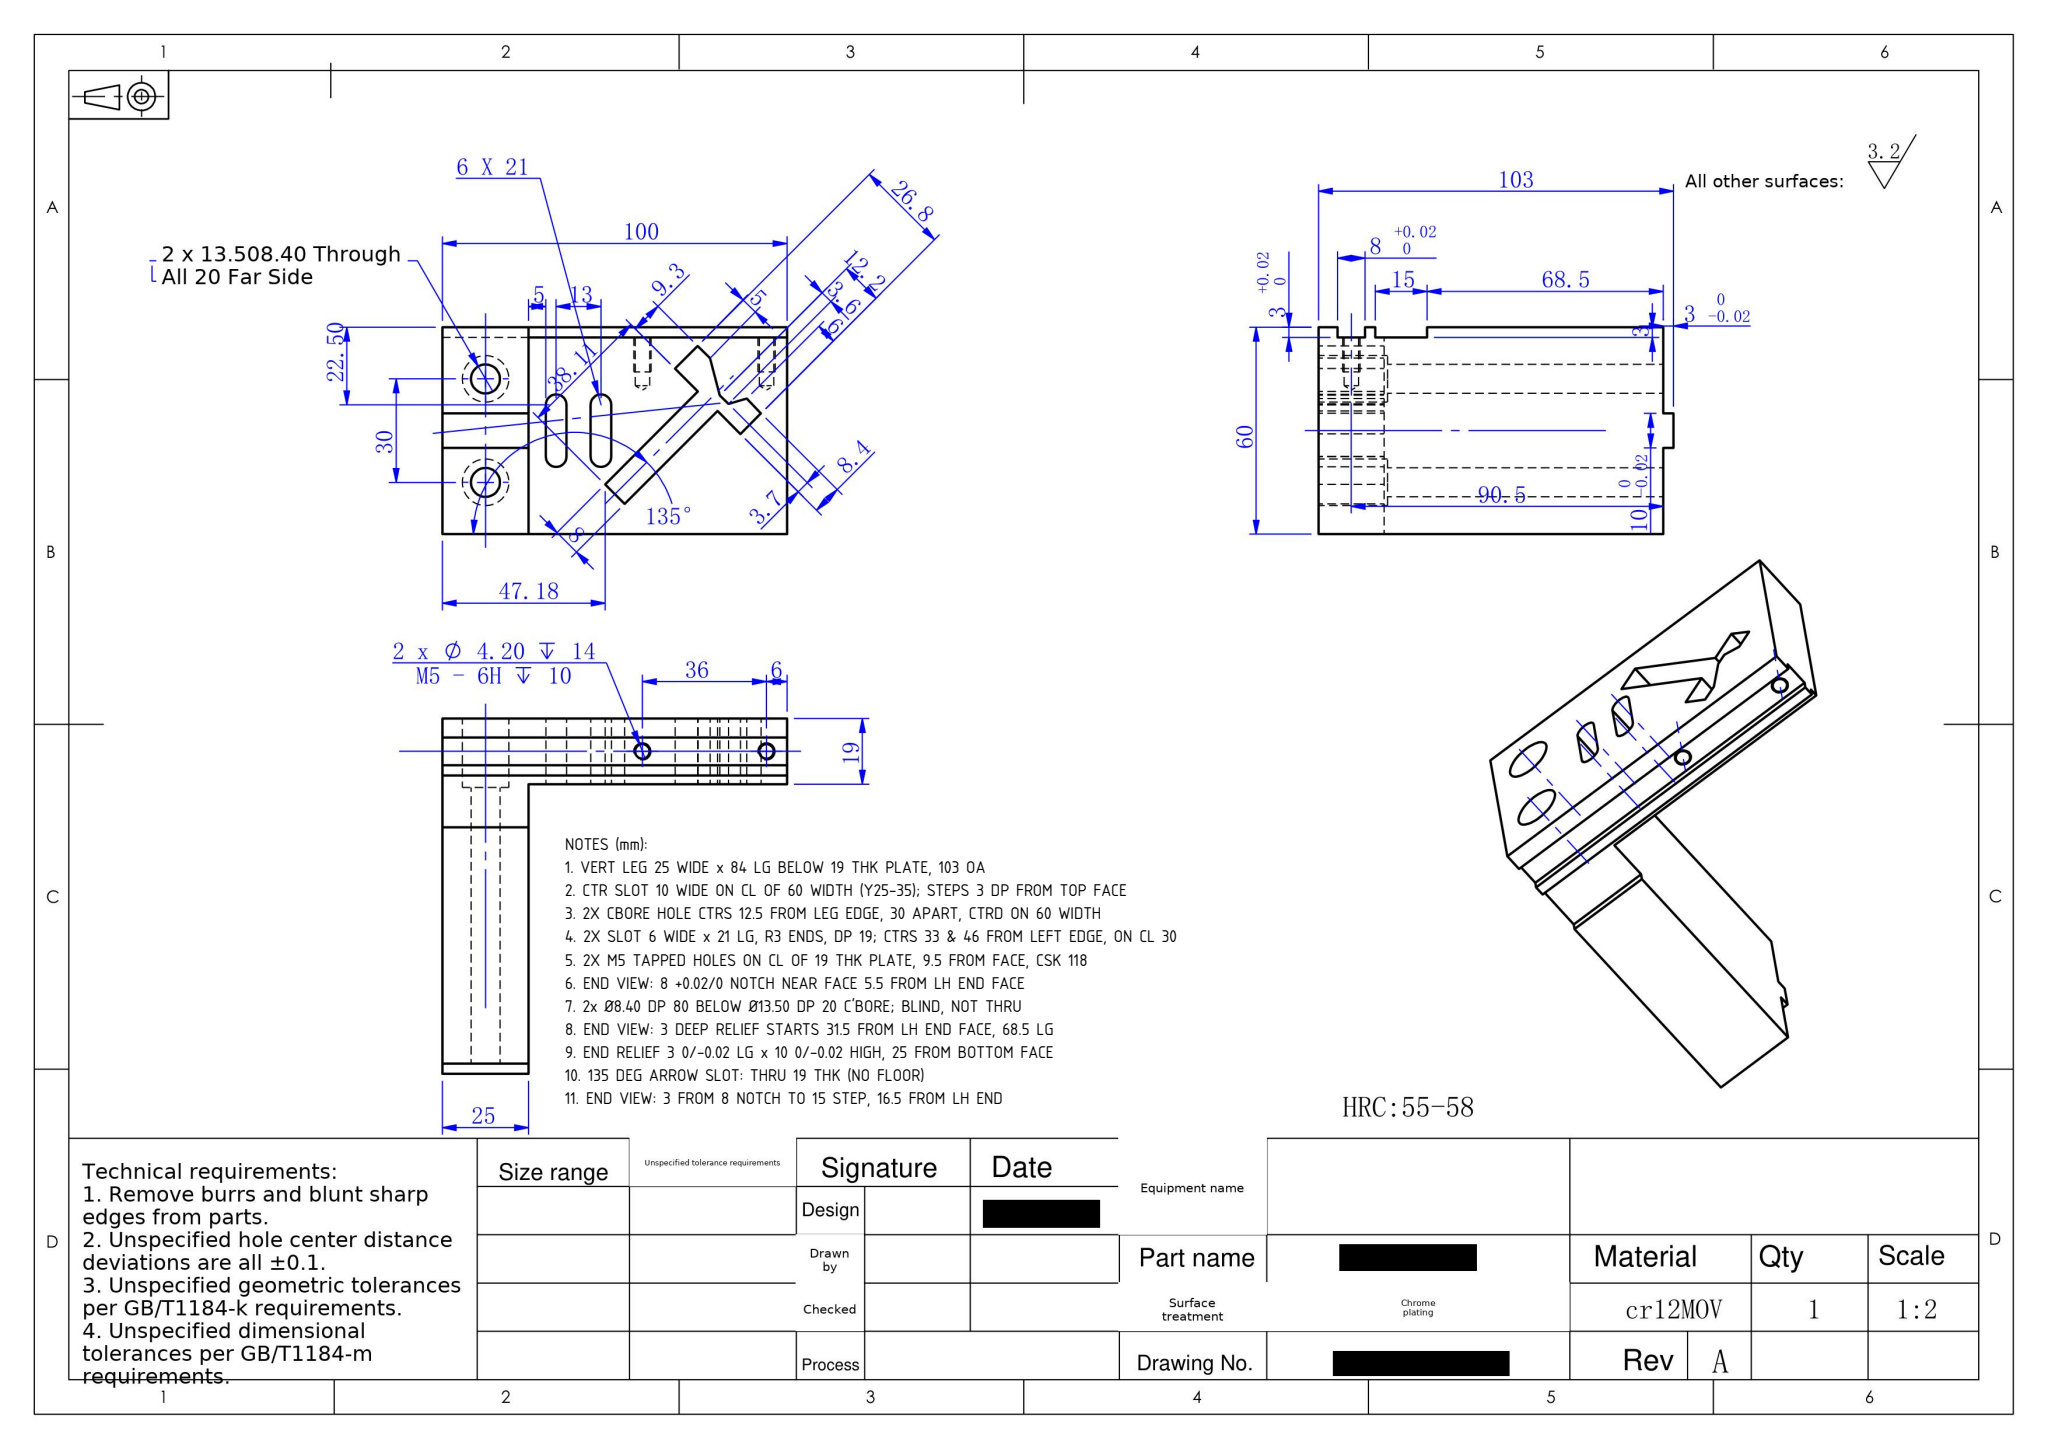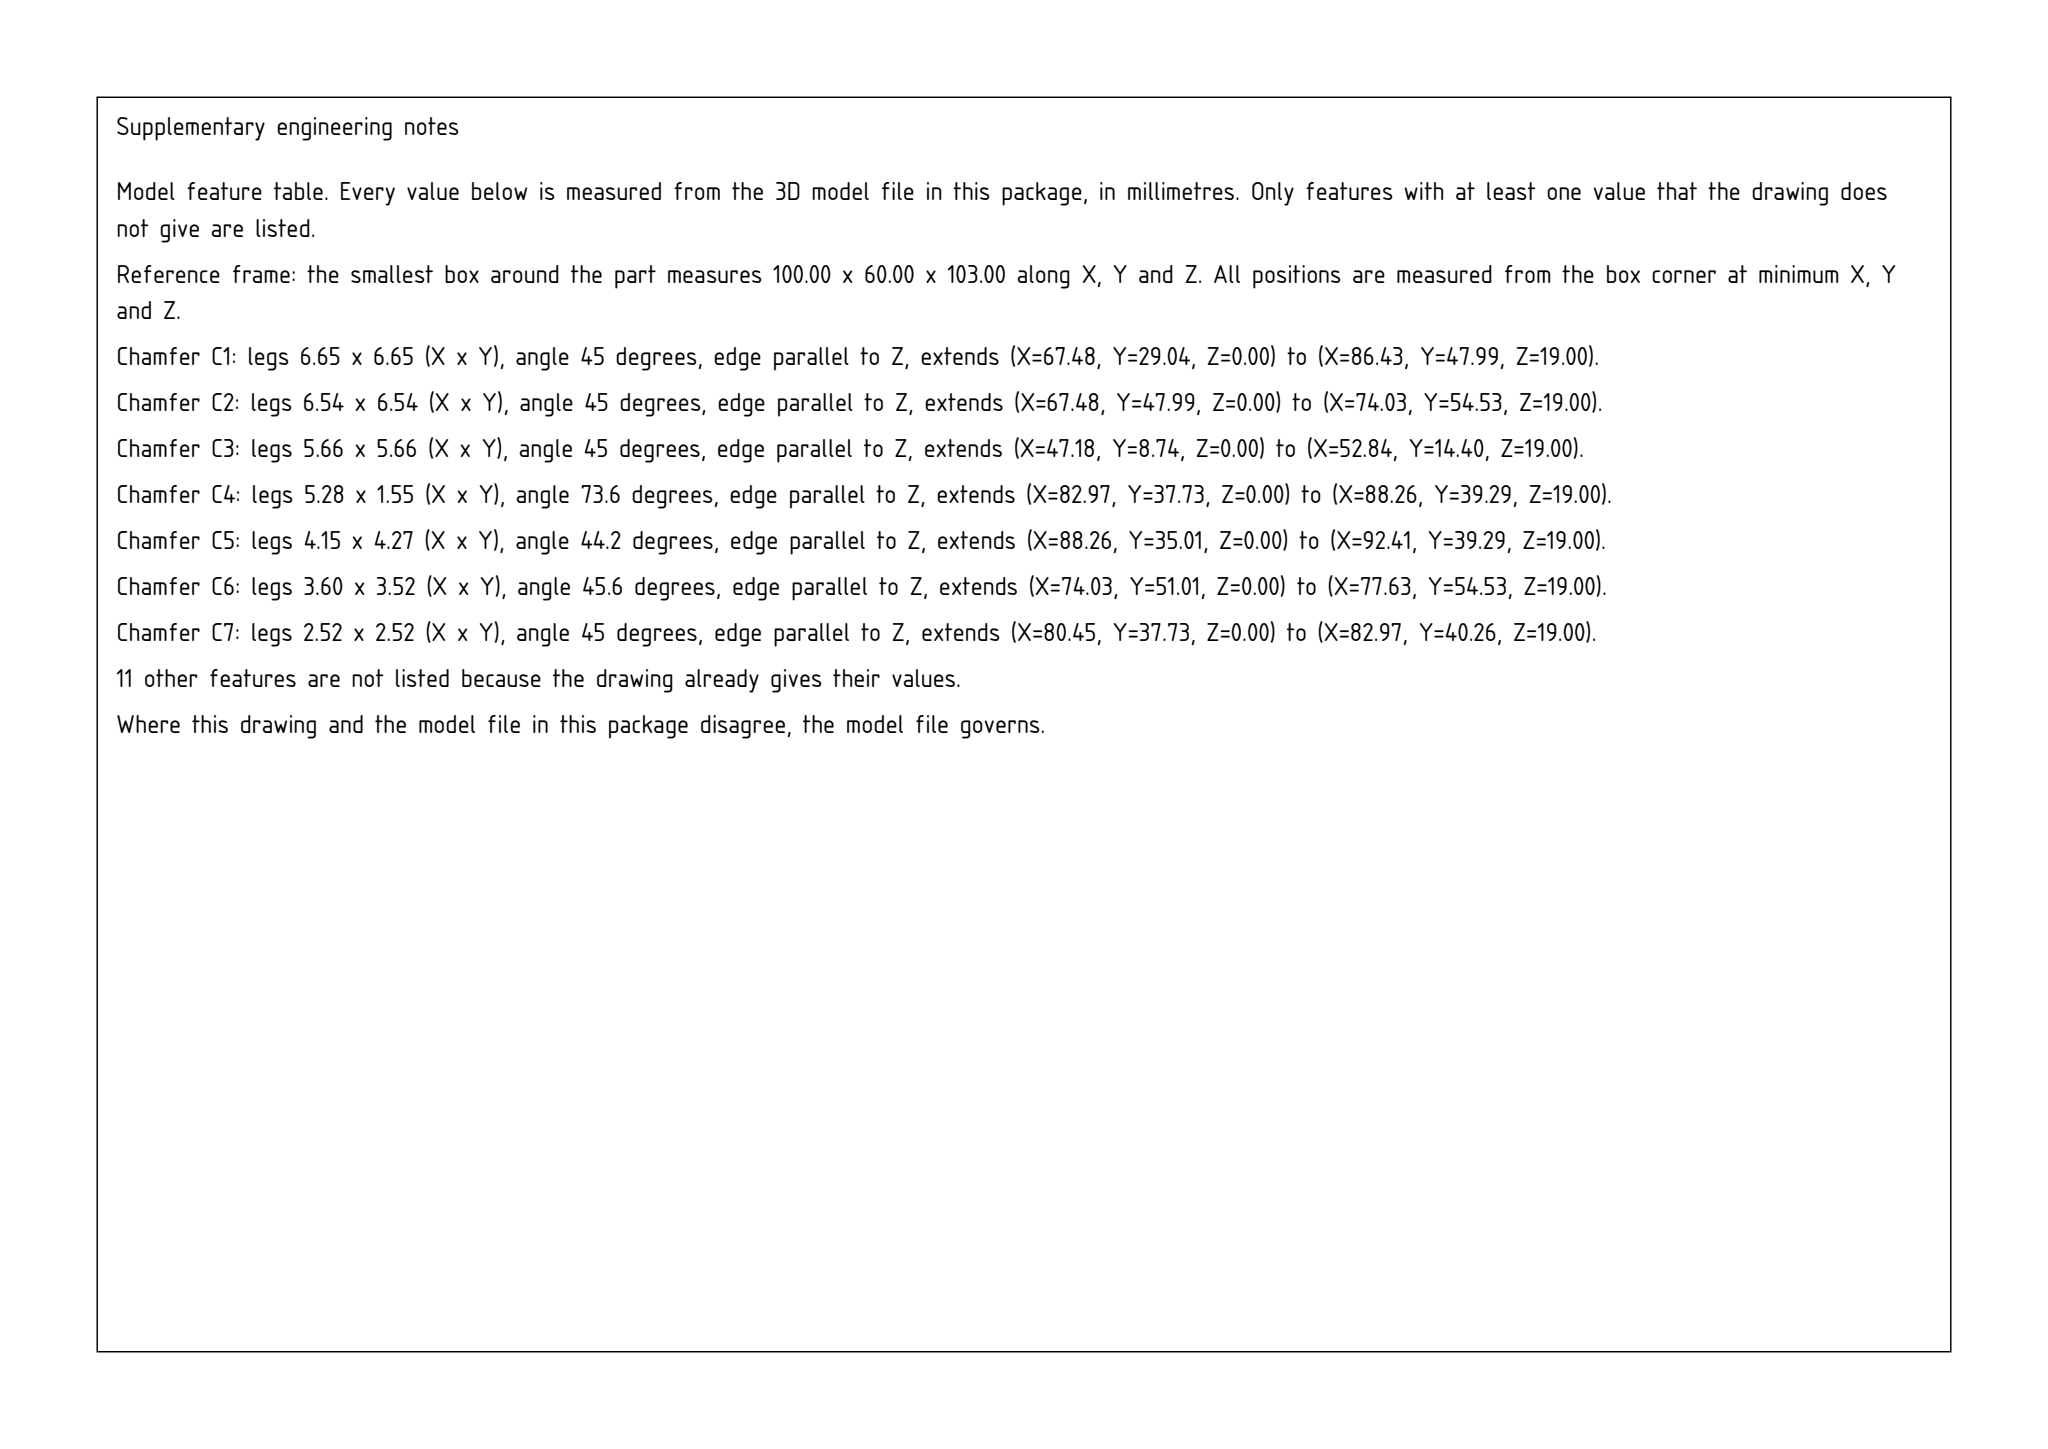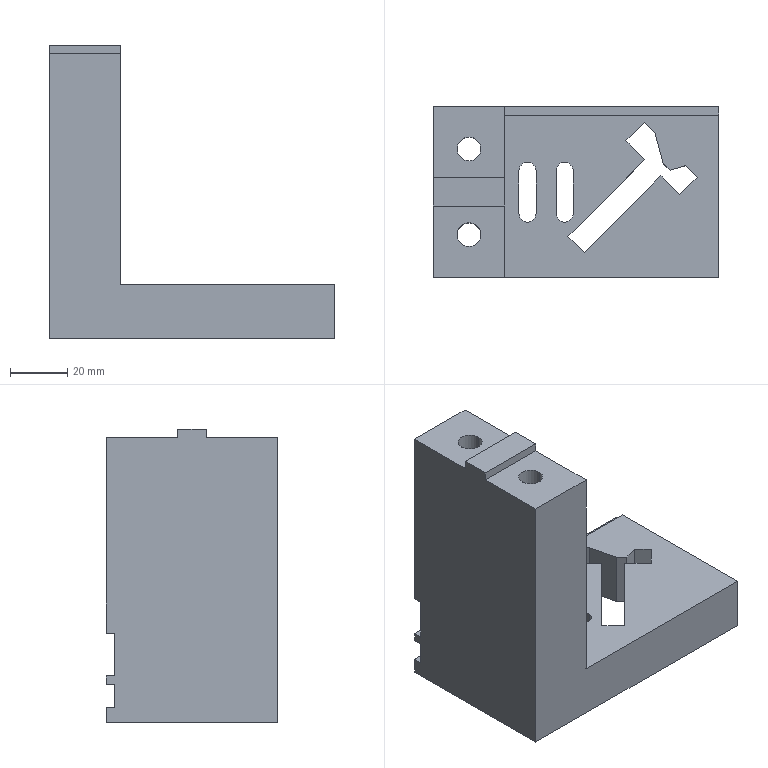Part | SolidWorks | mm | 1 solid | 58 faces | box 100 x 60 x 103 mm | volume 203290 mm3 | plane 38 | cylinder 16 | cone 4 | commonest cylinder face diameters 4.2 x4 13.5 x4 8.4 x4 6 x4
Drawing notes:
VERT LEG 25 WIDE x 84 LG BELOW 19 THK PLATE, 103 OA | from the solid: x-planes 0 & 25; z-planes 19 & 103; bbox z=103
CTR SLOT 10 WIDE ON CL OF 60 WIDTH (Y25-35); STEPS 3 DP FROM TOP FACE | from the solid: y-planes 25 & 35 (10 wide, CL 30); y-planes 57 & 60 (3 step)
2X CBORE HOLE CTRS 12.5 FROM LEG EDGE, 30 APART, CTRD ON 60 WIDTH | from the solid: O8.4/O13.5 z-cyls at x=12.5, y=15 & 45; bbox y=60
2X SLOT 6 WIDE x 21 LG, R3 ENDS, DP 19; CTRS 33 & 46 FROM LEFT EDGE, ON CL 30 | from the solid: O6 z-cyls L19 at x=33 & 46, y=22.5 & 37.5 (15 ctr + 6 = 21 lg)
2X M5 TAPPED HOLES ON CL OF 19 THK PLATE, 9.5 FROM FACE, CSK 118 | from the solid: O4.2 y-axis cyls L14 at z=9.5, x=58 & 94; cone 118 ref dia 4.2
END VIEW: 8 +0.02/0 NOTCH NEAR FACE 5.5 FROM LH END FACE | from the solid: z-planes at 5.5 and 13.5 (8 apart) = notch faces; LH end face z=0, overall 103
2x Ø8.40 DP 80 BELOW Ø13.50 DP 20 C'BORE; BLIND, NOT THRU | from the solid: cyl Ø13.5 len 20 and Ø8.4 len 80 coaxial at (12.5,15) & (12.5,45); total 100 < 103 length
END VIEW: 3 DEEP RELIEF STARTS 31.5 FROM LH END FACE, 68.5 LG | from the solid: y=57 face (3 below y=60 top) spans z=31.5 to z=100; 31.5+68.5=100, LH end z=0
END RELIEF 3 0/-0.02 LG x 10 0/-0.02 HIGH, 25 FROM BOTTOM FACE | from the solid: z-planes 100/103 (3) with y-planes 25/35 (10) at RH end
135 DEG ARROW SLOT: THRU 19 THK (NO FLOOR) | from the solid: Slot faces are non-axis-aligned; no z-plane between z=0 and z=19 bar bottom, so cut passes through full 19 plate thickness (z planes 0 and 19)
END VIEW: 3 FROM 8 NOTCH TO 15 STEP, 16.5 FROM LH END | from the solid: z planes 5.5, 13.5, 16.5: 5.5+8=13.5, +3=16.5, then 16.5+15=31.5, +68.5=100, +3=103
build123d program:
from build123d import *

# Parameters (mm, degrees)
SKETCH1_W                                       = 40
SKETCH1_H                                       = 60
BOSS_EXTRUDE1_DEPTH                             = 19
CUT_EXTRUDE1_DEPTH                              = 121.668
SKETCH6_W                                       = 19
SKETCH6_H                                       = 60
BOSS_EXTRUDE5_DEPTH                             = 35
SKETCH7_W                                       = 100
SKETCH7_H                                       = 60
BOSS_EXTRUDE6_DEPTH                             = 25
M8_HEX_SOCKET_HEAD_CAP_SCREW_CBORE1_D           = 8.4
M8_HEX_SOCKET_HEAD_CAP_SCREW_CBORE1_CBORE_D     = 13.5
M8_HEX_SOCKET_HEAD_CAP_SCREW_CBORE1_CBORE_DEPTH = 20
SKETCH10_W                                      = 25
SKETCH10_H                                      = 10
BOSS_EXTRUDE7_DEPTH                             = 3
CUT_EXTRUDE2_DEPTH                              = 202.606
SKETCH12_W                                      = 8
SKETCH12_H                                      = 3
CUT_EXTRUDE3_DEPTH                              = 157.241
M5_TAPPED_HOLE1_D                               = 4.2
M5_TAPPED_HOLE1_DEPTH                           = 14
M5_TAPPED_HOLE1_TIP                             = 1.262
SKETCH16_W                                      = 15
SKETCH16_H                                      = 3
CUT_EXTRUDE4_DEPTH                              = 157.241
CUT_EXTRUDE5_DEPTH                              = 193.593


with BuildPart() as part:
    # Sketch1 → Boss-Extrude1 (new body)
    with BuildSketch(Plane.XY):
        with Locations((-81.969, 31.662)):
            Rectangle(SKETCH1_W, SKETCH1_H)
    extrude(amount=BOSS_EXTRUDE1_DEPTH)

    # Sketch2 → Cut-Extrude1 (cut, through all)
    with BuildSketch(Plane.XY.offset(19)):
        Polygon((-94.485, 49.652), (-75.534, 30.701), (-69.562, 36.674), (-73.713, 40.947), (-78.997, 39.396), (-81.52, 41.919), (-84.336, 52.673), (-87.941, 56.196), align=None)
    extrude(amount=-CUT_EXTRUDE1_DEPTH, mode=Mode.SUBTRACT)

    # Sketch6 → Boss-Extrude5 (add)
    with BuildSketch(Plane.ZY.offset(101.969)):
        with Locations((9.5, 31.662)):
            Rectangle(SKETCH6_W, SKETCH6_H)
    extrude(amount=BOSS_EXTRUDE5_DEPTH)

    # Sketch7 → Boss-Extrude6 (add)
    with BuildSketch(Plane.ZY.offset(136.969)):
        with Locations((50, 31.662)):
            Rectangle(SKETCH7_W, SKETCH7_H)
    extrude(amount=BOSS_EXTRUDE6_DEPTH)

    # M8 Hex Socket Head Cap Screw CBORE1 (through all)
    with Locations(Plane(origin=(0, 0, 0), x_dir=(-1, 0, 0), z_dir=(0, 0, -1))):
        with Locations((149.469, 46.662), (149.469, 16.662)):
            CounterBoreHole(M8_HEX_SOCKET_HEAD_CAP_SCREW_CBORE1_D / 2, M8_HEX_SOCKET_HEAD_CAP_SCREW_CBORE1_CBORE_D / 2, M8_HEX_SOCKET_HEAD_CAP_SCREW_CBORE1_CBORE_DEPTH)

    # Sketch10 → Boss-Extrude7 (add)
    with BuildSketch(Plane.XY.offset(100)):
        with Locations((-149.469, 31.662)):
            Rectangle(SKETCH10_W, SKETCH10_H)
    extrude(amount=BOSS_EXTRUDE7_DEPTH)

    # Sketch11 → Cut-Extrude2 (cut, through all)
    with BuildSketch(Plane(origin=(0, 0, 0), x_dir=(-1, 0, 0), z_dir=(0, 0, -1))):
        Polygon((87.838, 43.005), (114.785, 16.058), (109.128, 10.401), (82.181, 37.348), align=None)
    extrude(amount=-CUT_EXTRUDE2_DEPTH, mode=Mode.SUBTRACT)

    # Sketch12 → Cut-Extrude3 (cut, through all)
    with BuildSketch(Plane.ZY.offset(161.969)):
        with Locations((9.5, 60.162)):
            Rectangle(SKETCH12_W, SKETCH12_H)
    extrude(amount=-CUT_EXTRUDE3_DEPTH, mode=Mode.SUBTRACT)

    # M5 Tapped Hole1
    with Locations(Plane(origin=(0, 58.662, 0), x_dir=(1, 0, 0), z_dir=(0, 1, 0))):
        with Locations((-103.969, -9.5), (-67.969, -9.5)):
            Hole(M5_TAPPED_HOLE1_D / 2, depth=M5_TAPPED_HOLE1_DEPTH)
            with Locations((0, 0, -(M5_TAPPED_HOLE1_DEPTH + M5_TAPPED_HOLE1_TIP / 2))):  # 118° drill point
                Cone(0, M5_TAPPED_HOLE1_D / 2, M5_TAPPED_HOLE1_TIP, mode=Mode.SUBTRACT)

    # Sketch16 → Cut-Extrude4 (cut, through all)
    with BuildSketch(Plane.ZY.offset(161.969)):
        with Locations((24, 60.162)):
            Rectangle(SKETCH16_W, SKETCH16_H)
    extrude(amount=-CUT_EXTRUDE4_DEPTH, mode=Mode.SUBTRACT)

    # Sketch17 → Cut-Extrude5 (cut, through all)
    with BuildSketch(Plane.XY.offset(19)):
        with BuildLine():
            Line((-125.969, 39.162), (-125.969, 24.162))
            ThreePointArc((-125.969, 24.162), (-128.969, 21.162), (-131.969, 24.162))
            Line((-131.969, 24.162), (-131.969, 39.162))
            ThreePointArc((-131.969, 39.162), (-128.969, 42.162), (-125.969, 39.162))
        make_face()
        with BuildLine():
            Line((-112.969, 39.162), (-112.969, 24.162))
            ThreePointArc((-112.969, 24.162), (-115.969, 21.162), (-118.969, 24.162))
            Line((-118.969, 24.162), (-118.969, 39.162))
            ThreePointArc((-118.969, 39.162), (-115.969, 42.162), (-112.969, 39.162))
        make_face()
    extrude(amount=-CUT_EXTRUDE5_DEPTH, mode=Mode.SUBTRACT)


solid = part.part